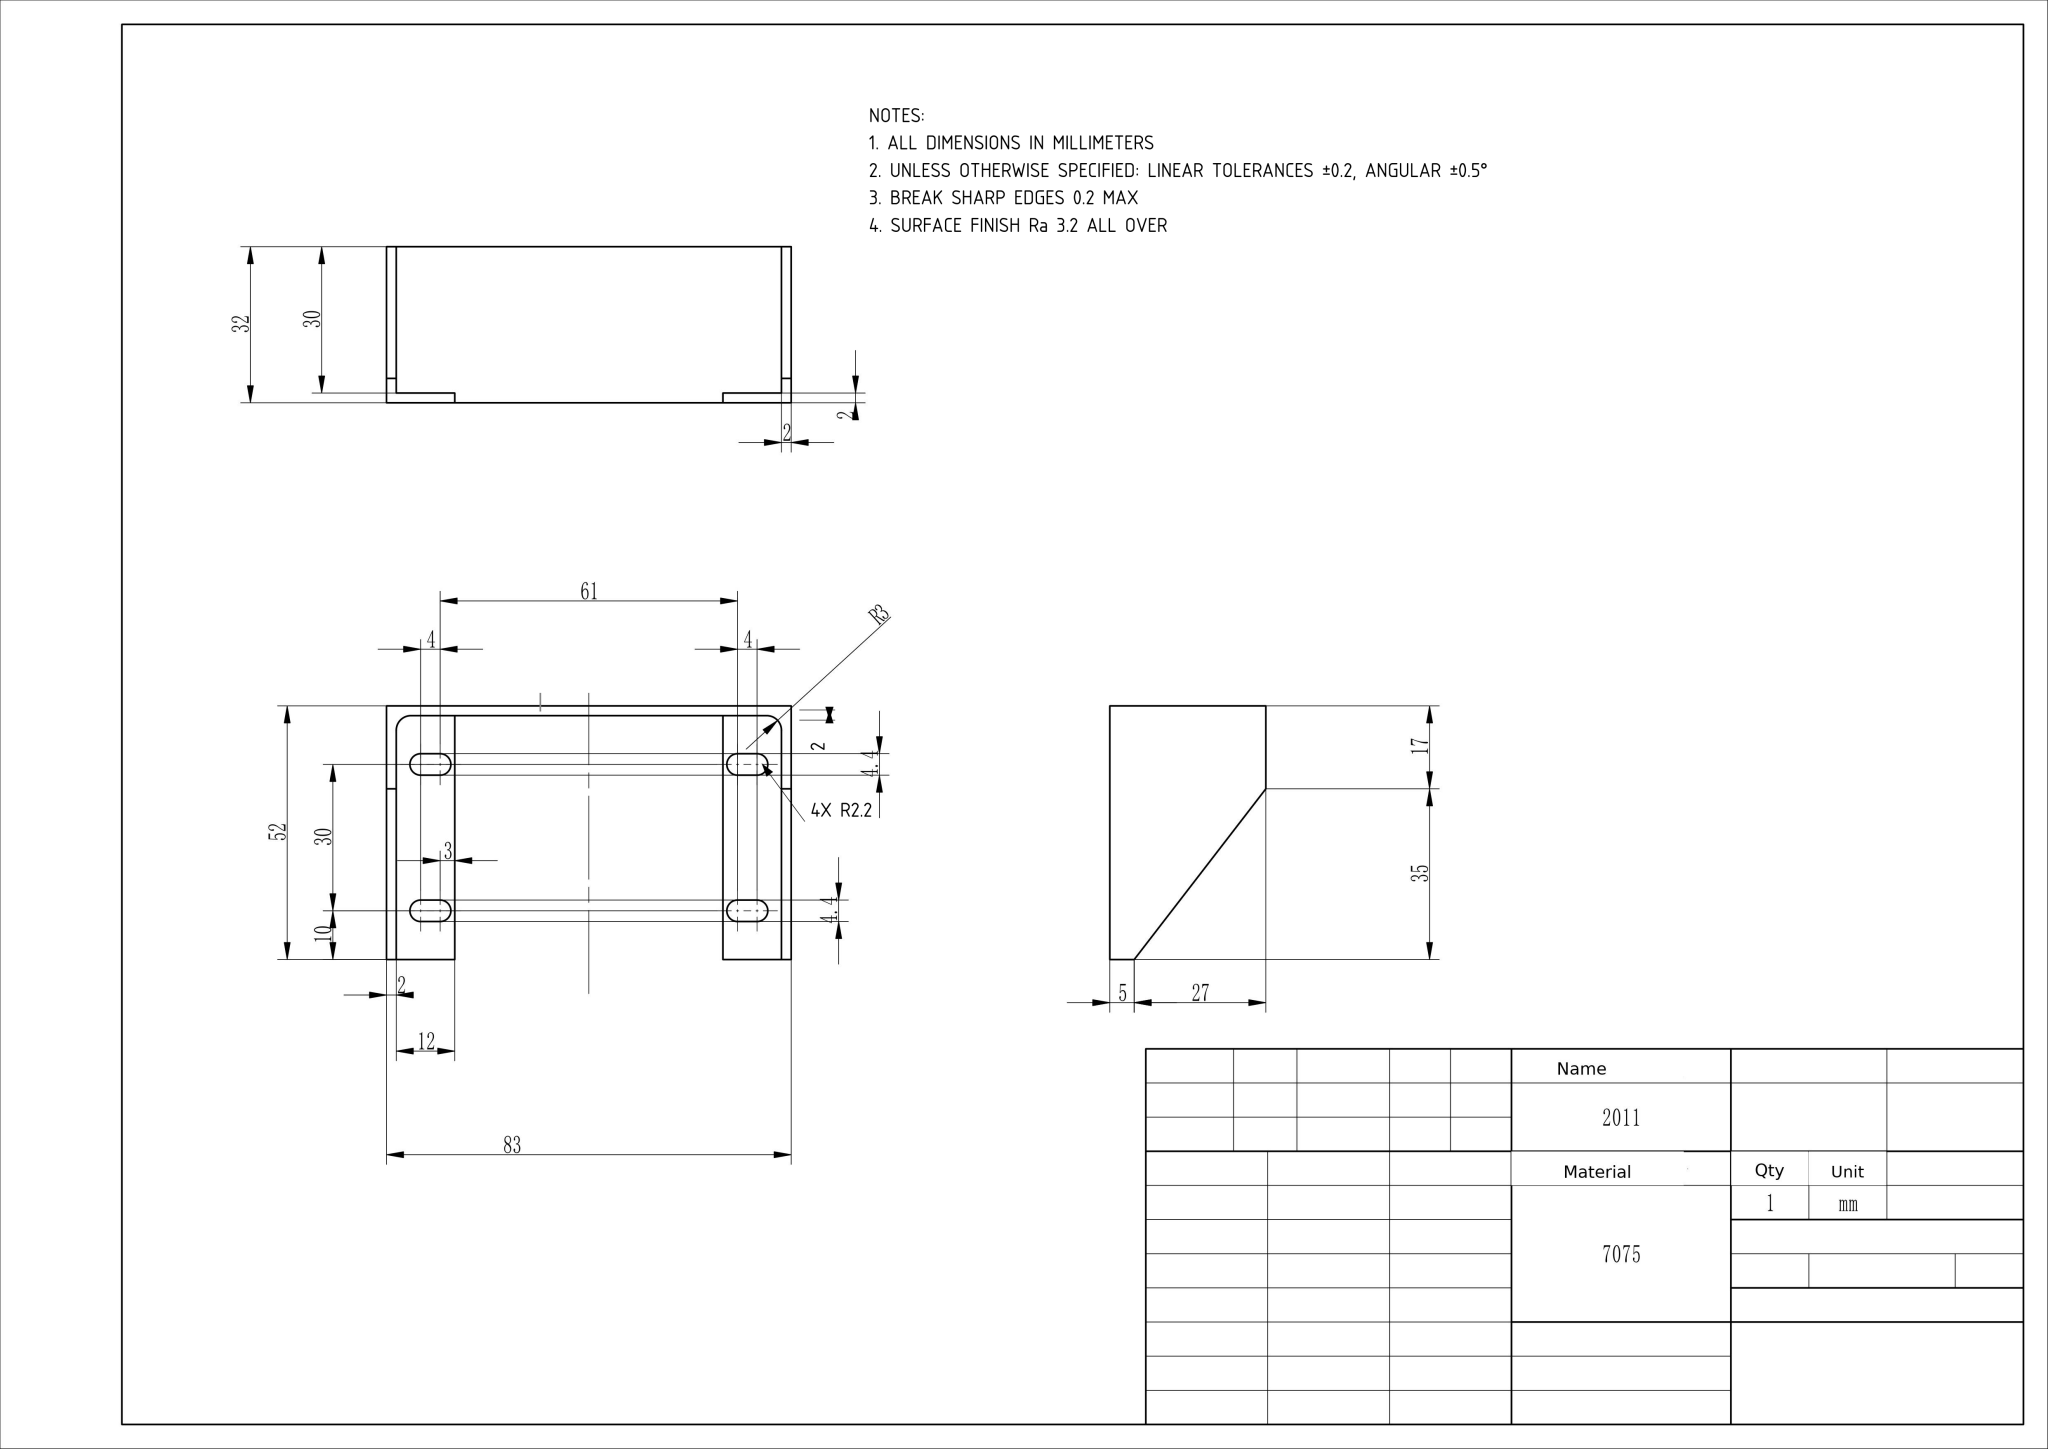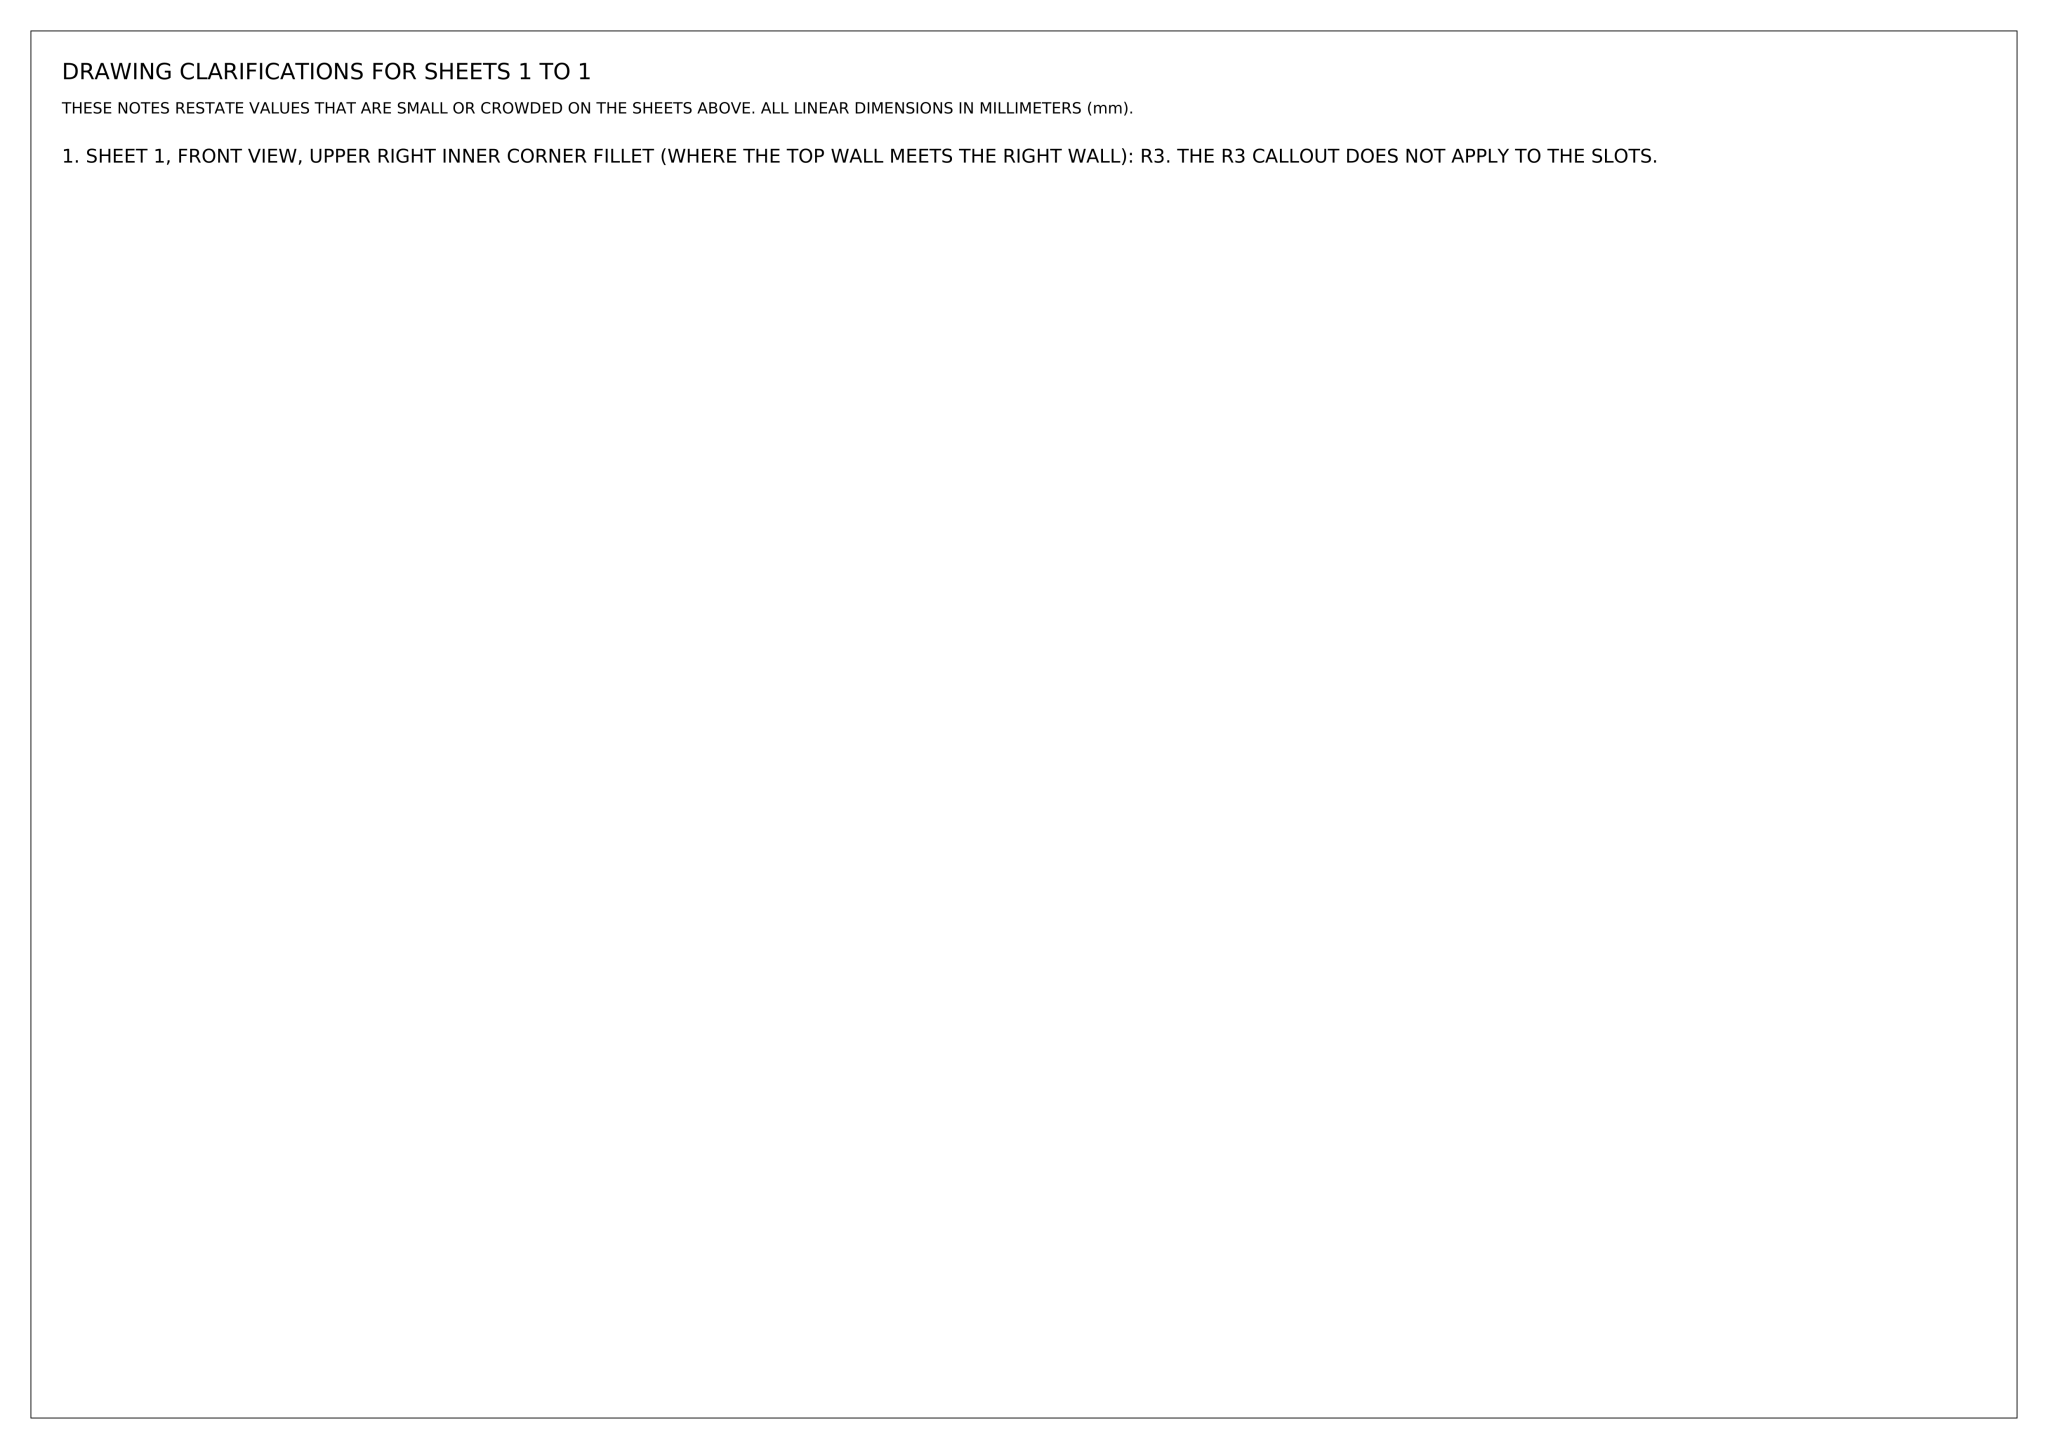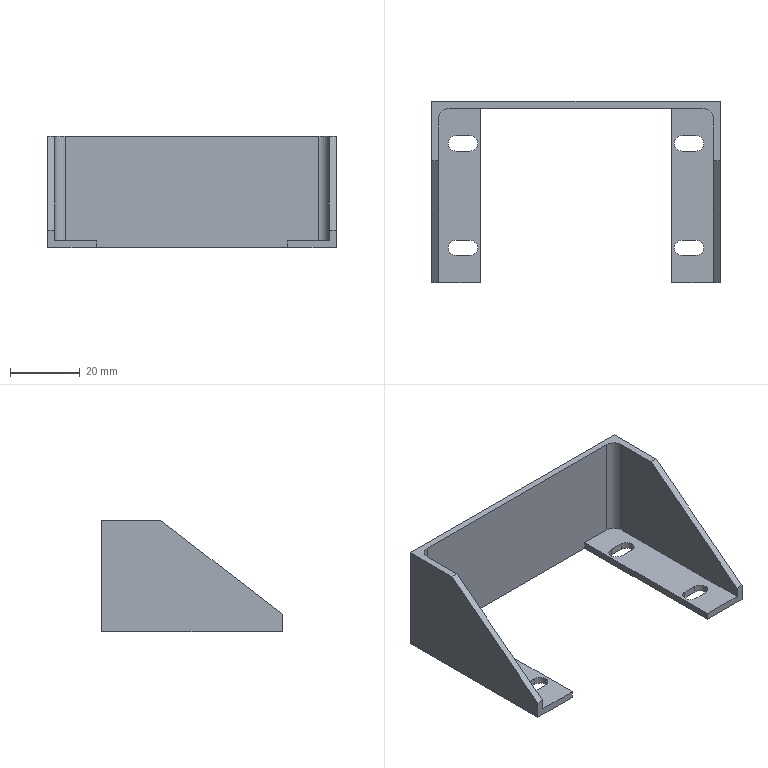Part | NX | mm | 1 solid | 34 faces | box 83 x 52 x 32 mm | volume 12075 mm3 | plane 24 | cylinder 10 | commonest cylinder face diameters 4.4 x8 6 x2